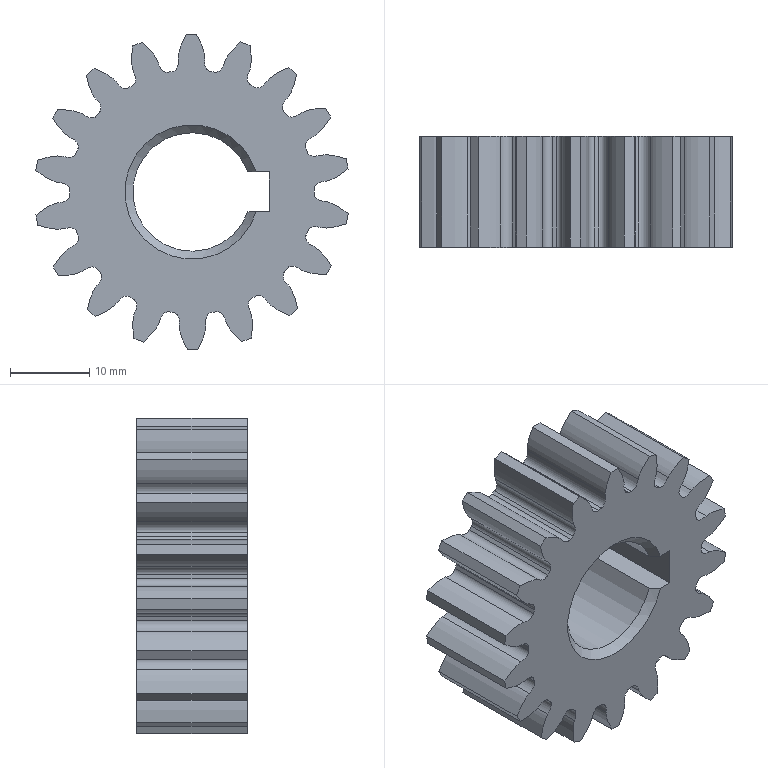Component | NX | CLHKJG_04_GEAR | 1 solid | 116 faces | volume 11130 mm3 | spline 90 | cylinder 19 | plane 5 | cone 2 | commonest cylinder face diameters 30.9 x18 15 x1